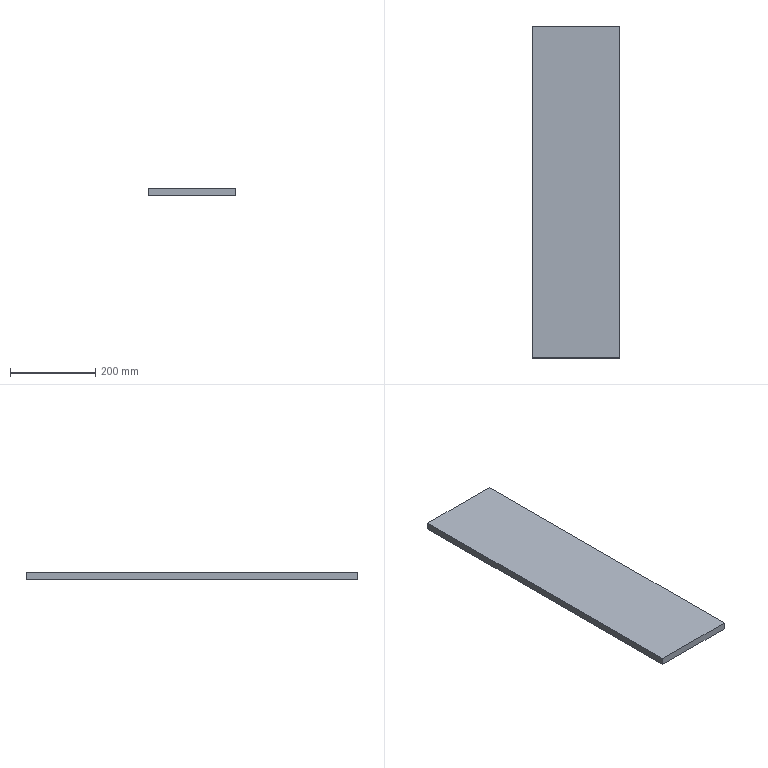Component | SolidWorks | Part37-1 | 1 solid | 6 faces | box 205 x 780 x 17 mm | volume 2718300 mm3 | plane 6
build123d program:
from build123d import *

# Parameters (mm, degrees)
SKETCH1_W           = 780
SKETCH1_H           = 205
BOSS_EXTRUDE1_DEPTH = 17


with BuildPart() as part:
    # Sketch1 → Boss-Extrude1 (new body)
    with BuildSketch(Plane.XY):
        Rectangle(SKETCH1_W, SKETCH1_H)
    extrude(amount=BOSS_EXTRUDE1_DEPTH)


solid = part.part

# Placed as in the assembly
solid = solid.moved(Location((-87.007, -16, -427), (0, 0, 90)))
STEP:
#1=COLOUR_RGB('',0.7922,0.8196,0.9333);
#2=FILL_AREA_STYLE_COLOUR('',#1);
#3=FILL_AREA_STYLE('',(#2));
#4=SURFACE_STYLE_FILL_AREA(#3);
#5=SURFACE_SIDE_STYLE('',(#4));
#6=SURFACE_STYLE_USAGE(.BOTH.,#5);
#7=PRESENTATION_STYLE_ASSIGNMENT((#6));
#8=CARTESIAN_POINT('',(0.61,14.724,-16.811));
#9=VERTEX_POINT('',#8);
#10=CARTESIAN_POINT('',(-7.461,14.724,-16.811));
#11=VERTEX_POINT('',#10);
#12=CARTESIAN_POINT('',(0.61,14.724,-16.811));
#13=DIRECTION('',(-1.,-0.,0.));
#14=VECTOR('',#13,39.37);
#15=LINE('',#12,#14);
#16=EDGE_CURVE('',#9,#11,#15,.T.);
#17=ORIENTED_EDGE('',*,*,#16,.T.);
#18=CARTESIAN_POINT('',(-7.461,14.724,-16.142));
#19=VERTEX_POINT('',#18);
#20=CARTESIAN_POINT('',(-7.461,14.724,-16.142));
#21=DIRECTION('',(0.,0.,-1.));
#22=VECTOR('',#21,39.37);
#23=LINE('',#20,#22);
#24=EDGE_CURVE('',#19,#11,#23,.T.);
#25=ORIENTED_EDGE('',*,*,#24,.F.);
#26=CARTESIAN_POINT('',(0.61,14.724,-16.142));
#27=VERTEX_POINT('',#26);
#28=CARTESIAN_POINT('',(0.61,14.724,-16.142));
#29=DIRECTION('',(-1.,-0.,0.));
#30=VECTOR('',#29,39.37);
#31=LINE('',#28,#30);
#32=EDGE_CURVE('',#27,#19,#31,.T.);
#33=ORIENTED_EDGE('',*,*,#32,.F.);
#34=CARTESIAN_POINT('',(0.61,14.724,-16.142));
#35=DIRECTION('',(0.,0.,-1.));
#36=VECTOR('',#35,39.37);
#37=LINE('',#34,#36);
#38=EDGE_CURVE('',#27,#9,#37,.T.);
#39=ORIENTED_EDGE('',*,*,#38,.T.);
#40=EDGE_LOOP('',(#17,#25,#33,#39));
#41=FACE_OUTER_BOUND('',#40,.T.);
#42=CARTESIAN_POINT('',(0.61,14.724,-16.142));
#43=DIRECTION('',(0.,-1.,0.));
#44=DIRECTION('',(0.,0.,1.));
#45=AXIS2_PLACEMENT_3D('',#42,#43,#44);
#46=PLANE('',#45);
#47=ADVANCED_FACE('',(#41),#46,.F.);
#48=CARTESIAN_POINT('',(-7.461,-15.984,-16.811));
#49=VERTEX_POINT('',#48);
#50=CARTESIAN_POINT('',(-7.461,-15.984,-16.811));
#51=DIRECTION('',(0.,-1.,0.));
#52=VECTOR('',#51,39.37);
#53=LINE('',#50,#52);
#54=EDGE_CURVE('',#11,#49,#53,.T.);
#55=ORIENTED_EDGE('',*,*,#54,.T.);
#56=CARTESIAN_POINT('',(-7.461,-15.984,-16.142));
#57=VERTEX_POINT('',#56);
#58=CARTESIAN_POINT('',(-7.461,-15.984,-16.142));
#59=DIRECTION('',(0.,0.,-1.));
#60=VECTOR('',#59,39.37);
#61=LINE('',#58,#60);
#62=EDGE_CURVE('',#57,#49,#61,.T.);
#63=ORIENTED_EDGE('',*,*,#62,.F.);
#64=CARTESIAN_POINT('',(-7.461,-15.984,-16.142));
#65=DIRECTION('',(0.,-1.,0.));
#66=VECTOR('',#65,39.37);
#67=LINE('',#64,#66);
#68=EDGE_CURVE('',#19,#57,#67,.T.);
#69=ORIENTED_EDGE('',*,*,#68,.F.);
#70=ORIENTED_EDGE('',*,*,#24,.T.);
#71=EDGE_LOOP('',(#55,#63,#69,#70));
#72=FACE_OUTER_BOUND('',#71,.T.);
#73=CARTESIAN_POINT('',(-7.461,-15.984,-16.142));
#74=DIRECTION('',(1.,0.,0.));
#75=DIRECTION('',(0.,0.,-1.));
#76=AXIS2_PLACEMENT_3D('',#73,#74,#75);
#77=PLANE('',#76);
#78=ADVANCED_FACE('',(#72),#77,.F.);
#79=CARTESIAN_POINT('',(0.61,-15.984,-16.811));
#80=VERTEX_POINT('',#79);
#81=CARTESIAN_POINT('',(0.61,-15.984,-16.811));
#82=DIRECTION('',(1.,0.,0.));
#83=VECTOR('',#82,39.37);
#84=LINE('',#81,#83);
#85=EDGE_CURVE('',#49,#80,#84,.T.);
#86=ORIENTED_EDGE('',*,*,#85,.T.);
#87=CARTESIAN_POINT('',(0.61,-15.984,-16.142));
#88=VERTEX_POINT('',#87);
#89=CARTESIAN_POINT('',(0.61,-15.984,-16.142));
#90=DIRECTION('',(0.,0.,-1.));
#91=VECTOR('',#90,39.37);
#92=LINE('',#89,#91);
#93=EDGE_CURVE('',#88,#80,#92,.T.);
#94=ORIENTED_EDGE('',*,*,#93,.F.);
#95=CARTESIAN_POINT('',(0.61,-15.984,-16.142));
#96=DIRECTION('',(1.,0.,0.));
#97=VECTOR('',#96,39.37);
#98=LINE('',#95,#97);
#99=EDGE_CURVE('',#57,#88,#98,.T.);
#100=ORIENTED_EDGE('',*,*,#99,.F.);
#101=ORIENTED_EDGE('',*,*,#62,.T.);
#102=EDGE_LOOP('',(#86,#94,#100,#101));
#103=FACE_OUTER_BOUND('',#102,.T.);
#104=CARTESIAN_POINT('',(0.61,-15.984,-16.142));
#105=DIRECTION('',(-0.,1.,0.));
#106=DIRECTION('',(0.,0.,-1.));
#107=AXIS2_PLACEMENT_3D('',#104,#105,#106);
#108=PLANE('',#107);
#109=ADVANCED_FACE('',(#103),#108,.F.);
#110=CARTESIAN_POINT('',(0.61,-15.984,-16.811));
#111=DIRECTION('',(-0.,1.,0.));
#112=VECTOR('',#111,39.37);
#113=LINE('',#110,#112);
#114=EDGE_CURVE('',#80,#9,#113,.T.);
#115=ORIENTED_EDGE('',*,*,#114,.T.);
#116=ORIENTED_EDGE('',*,*,#38,.F.);
#117=CARTESIAN_POINT('',(0.61,-15.984,-16.142));
#118=DIRECTION('',(-0.,1.,0.));
#119=VECTOR('',#118,39.37);
#120=LINE('',#117,#119);
#121=EDGE_CURVE('',#88,#27,#120,.T.);
#122=ORIENTED_EDGE('',*,*,#121,.F.);
#123=ORIENTED_EDGE('',*,*,#93,.T.);
#124=EDGE_LOOP('',(#115,#116,#122,#123));
#125=FACE_OUTER_BOUND('',#124,.T.);
#126=CARTESIAN_POINT('',(0.61,-15.984,-16.142));
#127=DIRECTION('',(-1.,-0.,0.));
#128=DIRECTION('',(0.,0.,1.));
#129=AXIS2_PLACEMENT_3D('',#126,#127,#128);
#130=PLANE('',#129);
#131=ADVANCED_FACE('',(#125),#130,.F.);
#132=ORIENTED_EDGE('',*,*,#32,.T.);
#133=ORIENTED_EDGE('',*,*,#68,.T.);
#134=ORIENTED_EDGE('',*,*,#99,.T.);
#135=ORIENTED_EDGE('',*,*,#121,.T.);
#136=EDGE_LOOP('',(#132,#133,#134,#135));
#137=FACE_OUTER_BOUND('',#136,.T.);
#138=CARTESIAN_POINT('',(-3.425,-0.6299,-16.142));
#139=DIRECTION('',(0.,0.,-1.));
#140=DIRECTION('',(0.,-1.,0.));
#141=AXIS2_PLACEMENT_3D('',#138,#139,#140);
#142=PLANE('',#141);
#143=ADVANCED_FACE('',(#137),#142,.F.);
#144=ORIENTED_EDGE('',*,*,#16,.F.);
#145=ORIENTED_EDGE('',*,*,#114,.F.);
#146=ORIENTED_EDGE('',*,*,#85,.F.);
#147=ORIENTED_EDGE('',*,*,#54,.F.);
#148=EDGE_LOOP('',(#144,#145,#146,#147));
#149=FACE_OUTER_BOUND('',#148,.T.);
#150=CARTESIAN_POINT('',(-3.425,-0.6299,-16.811));
#151=DIRECTION('',(0.,0.,-1.));
#152=DIRECTION('',(0.,-1.,0.));
#153=AXIS2_PLACEMENT_3D('',#150,#151,#152);
#154=PLANE('',#153);
#155=ADVANCED_FACE('',(#149),#154,.T.);
#156=CLOSED_SHELL('',(#47,#78,#109,#131,#143,#155));
#157=MANIFOLD_SOLID_BREP('',#156);
#158=STYLED_ITEM('',(#7),#157);
#159=PRESENTATION_LAYER_ASSIGNMENT('','',(#158));
#160=(LENGTH_UNIT()NAMED_UNIT(*)SI_UNIT($,.METRE.));
#161=LENGTH_MEASURE_WITH_UNIT(LENGTH_MEASURE(0.0254),#160);
#162=DIMENSIONAL_EXPONENTS(1.,0.,0.,0.,0.,0.,0.);
#163=(CONVERSION_BASED_UNIT('',#161)LENGTH_UNIT()NAMED_UNIT(#162));
#164=UNCERTAINTY_MEASURE_WITH_UNIT(LENGTH_MEASURE(0.00001),#163,'','');
#165=(NAMED_UNIT(*)PLANE_ANGLE_UNIT()SI_UNIT($,.RADIAN.));
#166=(NAMED_UNIT(*)SI_UNIT($,.STERADIAN.)SOLID_ANGLE_UNIT());
#167=(GEOMETRIC_REPRESENTATION_CONTEXT(3)GLOBAL_UNCERTAINTY_ASSIGNED_CONTEXT((#164))GLOBAL_UNIT_ASSIGNED_CONTEXT((#163,#165,#166))REPRESENTATION_CONTEXT('',''));
#168=MECHANICAL_DESIGN_GEOMETRIC_PRESENTATION_REPRESENTATION('',(#158),#167);
#169=CARTESIAN_POINT('',(0.,0.,0.));
#170=DIRECTION('',(0.,0.,1.));
#171=DIRECTION('',(1.,0.,0.));
#172=AXIS2_PLACEMENT_3D('',#169,#170,#171);
#173=(LENGTH_UNIT()NAMED_UNIT(*)SI_UNIT($,.METRE.));
#174=LENGTH_MEASURE_WITH_UNIT(LENGTH_MEASURE(0.0254),#173);
#175=DIMENSIONAL_EXPONENTS(1.,0.,0.,0.,0.,0.,0.);
#176=(CONVERSION_BASED_UNIT('',#174)LENGTH_UNIT()NAMED_UNIT(#175));
#177=UNCERTAINTY_MEASURE_WITH_UNIT(LENGTH_MEASURE(0.00001),#176,'','');
#178=(NAMED_UNIT(*)PLANE_ANGLE_UNIT()SI_UNIT($,.RADIAN.));
#179=(NAMED_UNIT(*)SI_UNIT($,.STERADIAN.)SOLID_ANGLE_UNIT());
#180=(GEOMETRIC_REPRESENTATION_CONTEXT(3)GLOBAL_UNCERTAINTY_ASSIGNED_CONTEXT((#177))GLOBAL_UNIT_ASSIGNED_CONTEXT((#176,#178,#179))REPRESENTATION_CONTEXT('',''));
#181=ADVANCED_BREP_SHAPE_REPRESENTATION('',(#157,#172),#180);